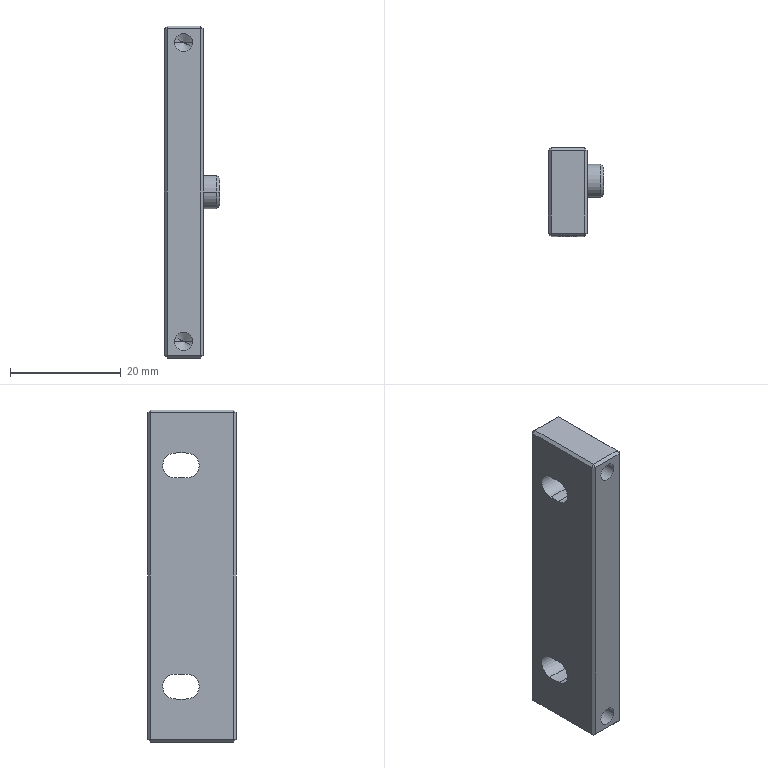CAM job | Mastercam | mm | 13 operations | part box 10 x 16 x 60
1. Facing | 24 - 100 平铣刀
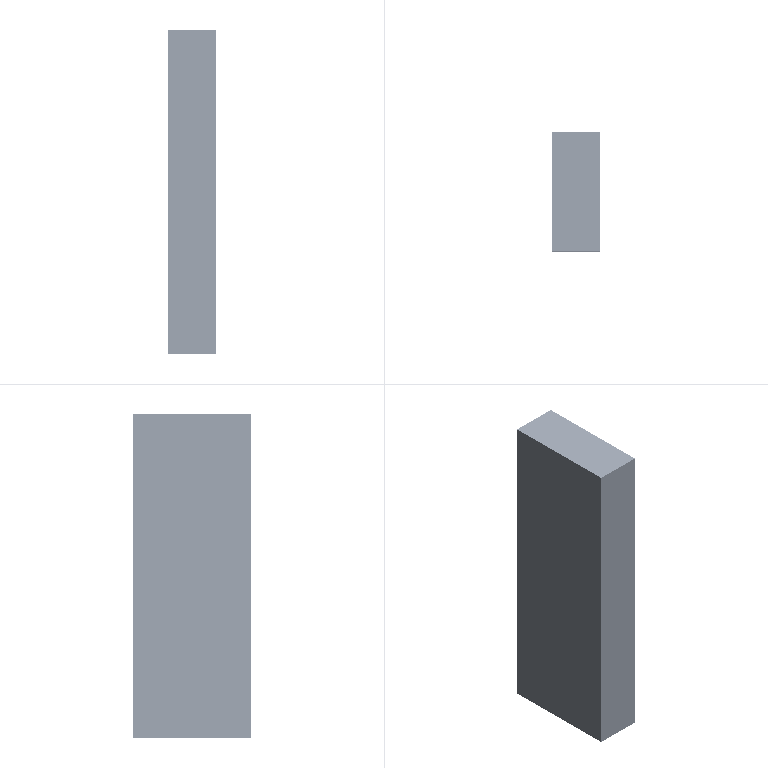2. Contour (Ramp) | 10 - 10 平铣刀
3. Contour (2D) | 10 - 10 平铣刀
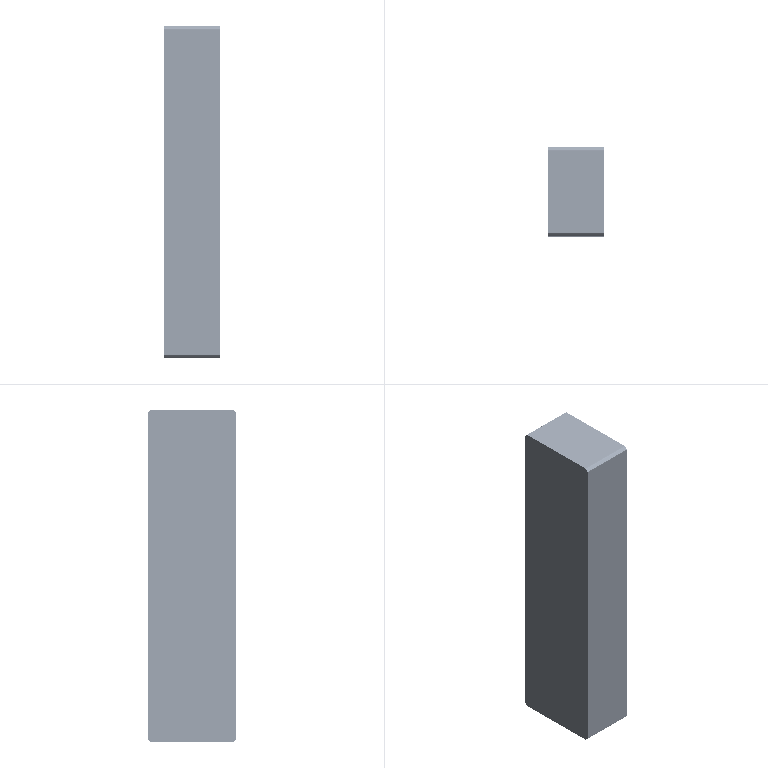4. Contour (Ramp) | 3 - 3 平铣刀
5. Contour (Ramp) | 3 - 3 平铣刀
6. Contour (2D chamfer) | 7 - 6 倒角刀
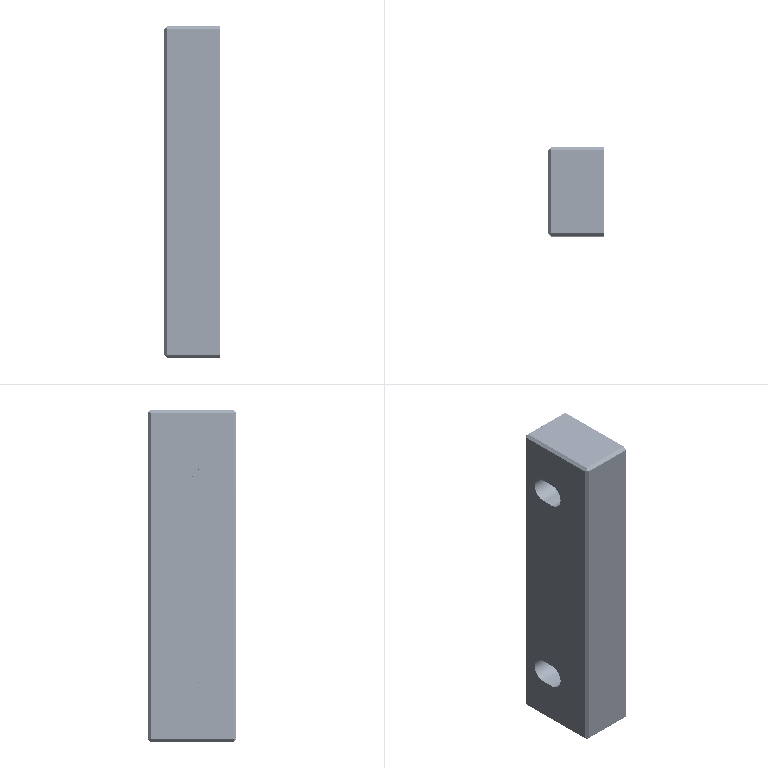7. Contour (2D chamfer) | 7 - 6 倒角刀
8. Facing | 24 - 100 平铣刀
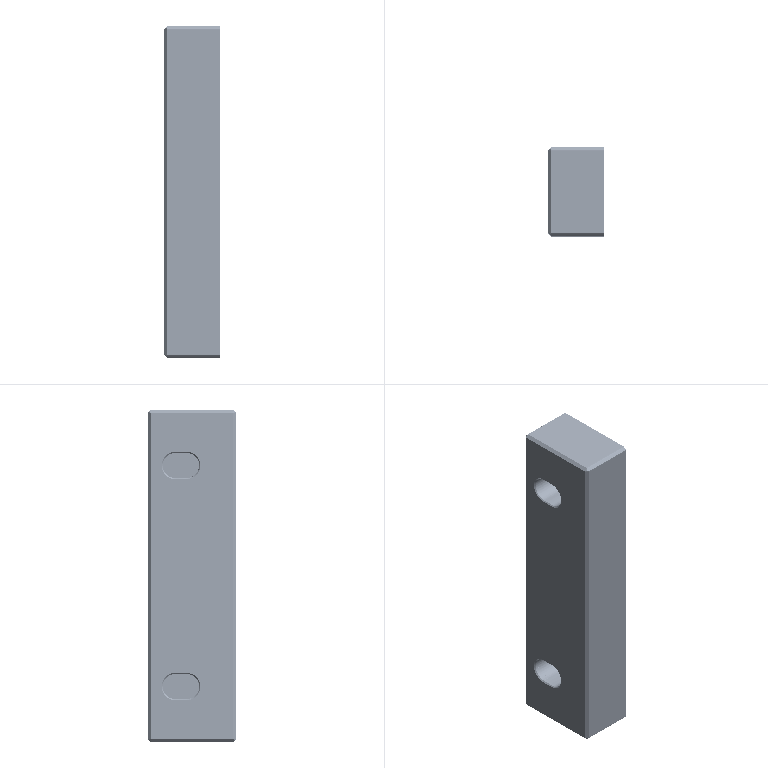9. 2D High Speed (2D Area Mill) | 10 - 10 平铣刀
10. Contour (2D) | 10 - 10 平铣刀
11. Contour (2D chamfer) | 7 - 6 倒角刀
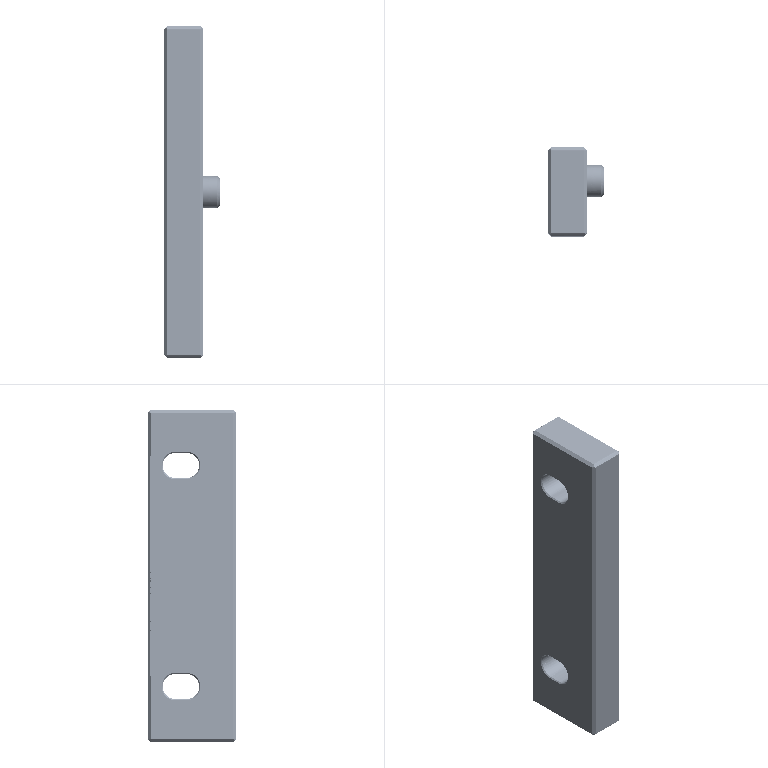12. Contour (2D chamfer) | 7 - 6 倒角刀
13. Drill/Counterbore | 7 - 6 倒角刀